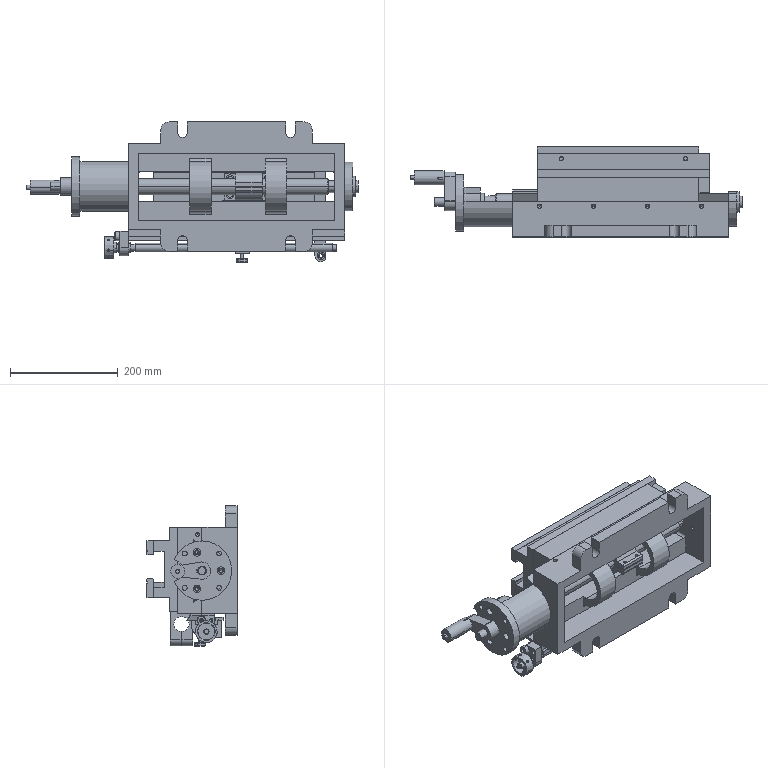Assembly | SolidWorks | mm | 25 component files | 25 solids | 853 faces | box 615 x 167 x 260 mm | volume 6916698 mm3 | cylinder 394 | plane 286 | cone 173 | commonest cylinder face diameters 6.8 x72 9 x54 14 x52 5 x27 8.5 x16 30 x14 10 x12 20 x12
Bill of materials:
10Pin | 1 |  | Stepped cylindrical pin: long slender shank, a short larger-diameter collar, a narrow groove/neck, then a short end section with a chamfered tip.
11HandleSleeve | 1 |  | Cylindrical tube/sleeve with a single axial slot starting at one end and ending in a rounded closed end.
13LargeKnurledNut | 1 |  | Cylindrical collar/hub with a smaller-diameter boss sticking out from one face, a central through bore, and several radial holes in the outer cylindrical surface.
14Washer | 1 |  | Flat annular ring (washer-like) with a rectangular cross-section and chamfered outer edges.
15LeadScrewPlate | 1 |  | Thick plate/block with a profile that is square at one end and fully rounded at the other, with one large through hole near the rounded end, two smaller through holes near the square end, and one chamfered corner.
17SmallKnurledNut | 1 |  | Thick-walled cylindrical spacer/bushing with chamfered outer edges at both ends and a chamfered or stepped bore edge.
19Insert | 1 |  | Long, thin flat strip or wedge with slightly tapered thickness along its length and angled ends, giving a parallelogram outline in one view.
1CopperSleeve | 1 |  | Flanged cylindrical bushing: a hollow cylindrical body with a larger-diameter flange at one end, chamfered edges, and a small step/relief next to the flange.
21MicrometerFrame | 1 |  | Elongated flat arm/bracket with a stepped profile. It has two small through holes, a side notch, a widened end section with a large through bore, a slit running from the bore to the end edge, and a small hole at the rounded opposite edge.
24FixtureBase | 1 |  | Rectangular plate with two parallel raised ribs/rails on one side, giving an E-like cross-section. It has a shallow rectangular pocket and a pattern of through holes in two sizes on the face.
25ClampingGuidePlate | 1 |  | Long, thin rectangular flat bar with two small holes or recesses near its ends on the top face.
27RightPressurePlate | 1 |  | Long rectangular bar with three evenly spaced holes through its side face and a small rectangular notch/step on one edge, visible in the end view.
29SlideSeat | 1 |  | Long rectangular block. One long side face has a stepped profile with a central rectangular channel and angled (dovetail-like) edges. It has a pattern of small holes on its faces.
2SemicircularSupportPlate | 1 |  | Thick disc-shaped plate with one straight flat side that has a small raised rectangular tab. It has a large central through-bore and three smaller through-holes.
30PressureBlock | 1 |  | Rectangular block with two countersunk through-holes side by side.
31FixedGuideRail | 1 |  | Long straight bar with a stepped cross-section: a wider base flange with a narrower raised rib on top. One upper edge of the rib is chamfered. A row of evenly spaced holes runs along the top.
32FineAdjustmentLeadScrew | 1 |  | Long slender stepped cylindrical shaft. One end has several reduced-diameter steps and a thin collar or ring. The other end has a short reduced-diameter journal.
33KnurledScrew | 1 |  | Headed pin: a short wide round disc head with a slender cylindrical shank in the centre. Both ends have small chamfers.
34Slider | 1 |  | Block-shaped bracket with a U-shaped top: two raised end lugs with paired holes. It has a large transverse through-bore, a central vertical hole with a slot across it, a smaller side hole, and one corner of the lower side cut at an angle.
36LeadScrewNut | 1 |  | Split-clamp style housing: a cylindrical boss with a large through-bore, a slotted projecting tab with two holes, and a perpendicular rectangular flange with four through-holes.
3LeadScrew | 1 |  | Long stepped cylindrical shaft. A main cylindrical section has a short reduced-diameter journal at one end. The other end has smaller stepped diameters and a thin collar.
4Base | 1 |  | Long rectangular frame-like housing with an open central window. It has two internal saddle-shaped cradle features, a cylindrical boss extending from one end, slotted mounting tabs along the sides, and several small holes on the end and side faces.
6IndexingPlate | 1 |  | Round flange disc with a central cylindrical hub on one side. The hub has a through-bore. Eight smaller holes are spaced around the flange, and the rim has one semicircular notch.
7Handle | 1 |  | Crank-like lever: a tapered flat arm with a larger rounded end holding a keyed bore and a smaller rounded end holding a plain hole. A cylindrical rod projects perpendicular from the arm.
9LeftPressurePlate | 1 |  | Long, straight, solid bar with a roughly rectangular cross-section (about 3:1 height to thickness as rendered). Three round holes pass through the wide face and appear evenly spaced along the length, one near each end and one at the middle. Three of the four long edges are chamfered, and one side face has a small rectangular groove that appears to run along the bar's length near one edge.
Mates:
1. coincident | 4Base-1 plane at (0, 0, 0) dir (0, 0, 1) | assembly plane at (0, 0, 0) dir (0, 0, 1)
2. coincident | 4Base-1 plane at (0, 0, 0) dir (0, 1, 0) | assembly plane at (0, 0, 0) dir (0, 1, 0)
3. coincident | 4Base-1 plane at (0, 0, 0) dir (1, 0, 0) | assembly plane at (0, 0, 0) dir (1, 0, 0)
4. coincident | 29SlideSeat-1 face at (-4.717, 81, 0) dir (0, -1, 0) | 4Base-1 face at (-293.381, 81, 46) dir (0, 1, 0)
5. coincident | 29SlideSeat-1 face at (145.283, 110, 80) dir (0, 0, 1) | 4Base-1 face at (-200, 65, 80) dir (0, 0, 1)
6. concentric | 3LeadScrew-1 face at (-232, 65, 0) dir (1, 0, 0) r 15 | 4Base-1 face at (-260, 65, 0) dir (-1, 0, 0) r 17.5
7. concentric | 3LeadScrew-1 face at (-345, 65, 0) dir (1, 0, 0) r 8 | 6IndexingPlate-1 face at (-310, 65, 0) dir (1, 0, 0) r 11
8. coincident | 3LeadScrew-1 face at (-260, 65, 0) dir (-1, 0, 0) | 6IndexingPlate-1 face at (-260, 65, 0) dir (1, 0, 0)
9. concentric | 4Base-1 face at (-290, 74.059, 33.807) dir (-1, 0, 0) r 3.4 | 6IndexingPlate-1 face at (-305, 74.059, 33.807) dir (-1, 0, 0) r 4.5
10. coincident | 4Base-1 face at (-290, 0, 0) dir (-1, 0, 0) | 6IndexingPlate-1 face at (-290, 65, 0) dir (1, 0, 0)
11. concentric | 3LeadScrew-1 face at (-345, 65, 0) dir (1, 0, 0) r 8 | 7Handle-1 face at (-305, 65, 0) dir (-1, 0, 0) r 8
12. coincident | 3LeadScrew-1 face at (-317.243, 69.87, 2.362) dir (0, -0.02861, -0.9996) | 7Handle-1 face at (-305, 110.053, 1.212) dir (0, -0.02861, -0.9996)
13. coincident | 6IndexingPlate-1 face at (-305, 65, 0) dir (-1, 0, 0) | 7Handle-1 face at (-305, 109.982, -1.287) dir (1, 0, 0)
14. concentric | 10Pin-1 face at (-327, 109.982, -1.287) dir (-1, 0, 0) r 4 | 11HandleSleeve-1 face at (-332, 109.982, -1.287) dir (-1, 0, 0) r 4.25
15. concentric | 10Pin-1 face at (-292, 109.982, -1.287) dir (-1, 0, 0) r 5 | 7Handle-1 face at (-392.971, 109.982, -1.287) dir (1, 0, 0) r 6
16. distance | 11HandleSleeve-1 face at (-327, 109.982, -1.287) dir (1, 0, 0) | 7Handle-1 face at (-326, 109.982, -1.287) dir (-1, 0, 0)
17. distance | 6IndexingPlate-1 face at (-290, 65, 0) dir (1, 0, 0) | 10Pin-1 face at (-292, 109.982, -1.287) dir (1, 0, 0)
18. coincident | 24FixtureBase-1 face at (5.283, 110, 2.5) dir (0, -1, 0) | 29SlideSeat-1 face at (145.283, 110, 80) dir (0, 1, 0)
19. coincident | 24FixtureBase-1 face at (-154.717, 155, -75) dir (-1, 0, 0) | 29SlideSeat-1 face at (-154.717, 87.5, 0) dir (-1, 0, 0)
20. coincident | 24FixtureBase-1 face at (-154.717, 155, 80) dir (0, 0, 1) | 29SlideSeat-1 face at (145.283, 110, 80) dir (0, 0, 1)
21. concentric | 2SemicircularSupportPlate-1 face at (200, 65, 0) dir (1, 0, 0) r 15 | 3LeadScrew-1 face at (170, 65, 0) dir (1, 0, 0) r 11
22. concentric | 2SemicircularSupportPlate-1 face at (215.5, 30, 0) dir (1, 0, 0) r 4.5 | 4Base-1 face at (200, 30, 0) dir (1, 0, 0) r 3.4
23. concentric | 1CopperSleeve-1 face at (225.5, 65, 0) dir (-1, 0, 0) r 11 | 2SemicircularSupportPlate-1 face at (200, 65, 0) dir (1, 0, 0) r 15
24. coincident | 1CopperSleeve-1 face at (215.5, 65, 0) dir (-1, 0, 0) | 2SemicircularSupportPlate-1 face at (215.5, 65, 0) dir (1, 0, 0)
25. concentric | 13LargeKnurledNut-1 face at (-222, 57, -113) dir (1, 0, 0) r 5 | 32FineAdjustmentLeadScrew-1 face at (-222, 57, -113) dir (1, 0, 0) r 7
26. concentric | 14Washer-1 face at (-219, 57, -113) dir (1, 0, 0) r 7 | 32FineAdjustmentLeadScrew-1 face at (-222, 57, -113) dir (1, 0, 0) r 7
27. concentric | 15LeadScrewPlate-1 face at (-280, 57, -113) dir (1, 0, 0) r 7 | 32FineAdjustmentLeadScrew-1 face at (-222, 57, -113) dir (1, 0, 0) r 7
28. coincident | 21MicrometerFrame-1 face at (143.283, 110, 71) dir (0, 1, 0) | 24FixtureBase-1 face at (5.283, 110, 2.5) dir (0, -1, 0)
29. coincident | 21MicrometerFrame-1 face at (165.283, 124, -139) dir (1, 0, 0) | 24FixtureBase-1 face at (165.283, 155, -75) dir (1, 0, 0)
30. coincident | 21MicrometerFrame-1 face at (143.283, 124, -75) dir (0, 0, 1) | 24FixtureBase-1 face at (-154.717, 155, -75) dir (0, 0, -1)
31. coincident | 31FixedGuideRail-1 face at (-200, 77, -100) dir (0, 0, -1) | 34Slider-1 face at (497.191, 37, -100) dir (0, 0, 1)
32. coincident | 31FixedGuideRail-1 face at (-200, 77, -80) dir (0, 1, 0) | 34Slider-1 face at (497.191, 77, -100) dir (0, -1, 0)
33. concentric | 32FineAdjustmentLeadScrew-1 face at (-188, 57, -113) dir (1, 0, 0) r 8 | 34Slider-1 face at (23.191, 57, -113) dir (1, 0, 0) r 8
34. coincident | 30PressureBlock-1 face at (10.191, 33, -92) dir (0, 0, -1) | 34Slider-1 face at (10.191, 57, -92) dir (0, 0, 1)
35. coincident | 30PressureBlock-1 face at (23.191, 26, -86) dir (1, 0, 0) | 34Slider-1 face at (23.191, 29, -124) dir (1, 0, 0)
36. concentric | 30PressureBlock-1 face at (17.191, 34, -86) dir (0, 0, 1) r 3.75 | 34Slider-1 face at (17.191, 34, -92) dir (0, 0, 1) r 1.65
37. concentric | 36LeadScrewNut-1 face at (47.897, 65, 0) dir (1, 0, 0) r 15 | 3LeadScrew-1 face at (-232, 65, 0) dir (1, 0, 0) r 15
38. concentric | 33KnurledScrew-1 face at (10.191, 69, -100) dir (0, 0, -1) r 3 | 34Slider-1 face at (10.191, 69, -100) dir (0, 0, 1) r 3
39. coincident | 24FixtureBase-1 face at (173.283, 175, -31) dir (0, 0, 1) | 25ClampingGuidePlate-1 face at (-154.717, 155, -31) dir (0, 0, -1)
40. coincident | 24FixtureBase-1 face at (5.283, 155, 2.5) dir (0, 1, 0) | 25ClampingGuidePlate-1 face at (-154.717, 155, -31) dir (0, 1, 0)
41. coincident | 24FixtureBase-1 face at (-154.717, 155, -75) dir (-1, 0, 0) | 25ClampingGuidePlate-1 face at (-154.717, 145, -26.5) dir (-1, 0, 0)
42. coincident | 24FixtureBase-1 face at (173.283, 185, 55) dir (0, 0, 1) | 27RightPressurePlate-1 face at (145.283, 155, 55) dir (0, 0, 1)
43. coincident | 24FixtureBase-1 face at (-154.717, 155, -75) dir (-1, 0, 0) | 27RightPressurePlate-1 face at (-154.717, 161, 42) dir (-1, 0, 0)
44. coincident | 24FixtureBase-1 face at (5.283, 155, 2.5) dir (0, 1, 0) | 27RightPressurePlate-1 face at (145.283, 155, 55) dir (0, -1, 0)
45. coincident | 24FixtureBase-1 face at (5.283, 155, 2.5) dir (0, 1, 0) | 9LeftPressurePlate-1 face at (-4.717, 155, -32.5) dir (0, -1, 0)
46. coincident | 24FixtureBase-1 face at (173.283, 185, -50) dir (0, 0, -1) | 9LeftPressurePlate-1 face at (-154.717, 167, -50) dir (0, 0, -1)
47. coincident | 24FixtureBase-1 face at (-154.717, 155, -75) dir (-1, 0, 0) | 9LeftPressurePlate-1 face at (-154.717, 167, -50) dir (-1, 0, 0)
48. distance | 33KnurledScrew-1 face at (10.191, 69, -140) dir (0, 0, -1) | 34Slider-1 face at (10.191, 57, -124) dir (0, 0, -1)
49. coincident | 31FixedGuideRail-1 face at (-200, 77, -80) dir (0, 0, 1) | 4Base-1 face at (-200, 65, -80) dir (0, 0, -1)
50. concentric | 31FixedGuideRail-1 face at (150, 57, -140) dir (0, 0, 1) r 4.5 | 4Base-1 face at (150, 57, -80) dir (0, 0, -1) r 3.4
51. concentric | 31FixedGuideRail-1 face at (-150, 57, -140) dir (0, 0, 1) r 4.5 | 4Base-1 face at (-150, 57, -80) dir (0, 0, -1) r 3.4
52. coincident | 13LargeKnurledNut-1 face at (-222, 57, -113) dir (1, 0, 0) | 32FineAdjustmentLeadScrew-1 face at (-222, 57, -113) dir (-1, 0, 0)
53. coincident | 19Insert-1 face at (-200, 92.935, -80) dir (0, 0, 1) | 29SlideSeat-1 face at (145.283, 110, -80) dir (0, 0, -1)
54. coincident | 19Insert-1 edge at (-200, 65, -80) dir (1, 0, 0) | 4Base-1 edge at (-200, 65, -80) dir (1, 0, 0)
55. coincident | 19Insert-1 face at (-200, 92.935, -84) dir (-1, 0, 0) | 31FixedGuideRail-1 face at (-200, 57, -90) dir (-1, 0, 0)
56. concentric | 15LeadScrewPlate-1 face at (-280, 48, -92) dir (1, 0, 0) r 3.25 | 31FixedGuideRail-1 face at (-200, 48, -92) dir (-1, 0, 0) r 2.5
57. coincident | 15LeadScrewPlate-1 face at (-200, 57, -113) dir (1, 0, 0) | 31FixedGuideRail-1 face at (-200, 57, -90) dir (-1, 0, 0)
58. coincident | 15LeadScrewPlate-1 face at (-200, 57, -113) dir (1, 0, 0) | 32FineAdjustmentLeadScrew-1 face at (-200, 57, -113) dir (-1, 0, 0)
59. concentric | 15LeadScrewPlate-1 face at (-280, 66, -92) dir (1, 0, 0) r 3.25 | 17SmallKnurledNut-1 face at (-216, 66, -92) dir (1, 0, 0) r 3.4
60. coincident | 15LeadScrewPlate-1 face at (-216, 57, -113) dir (-1, 0, 0) | 17SmallKnurledNut-1 face at (-216, 66, -92) dir (1, 0, 0)
61. parallel | 36LeadScrewNut-1 face at (47.897, 25, -10) dir (0, 0, -1) | 4Base-1 face at (182, 47, -62) dir (0, 0, 1)